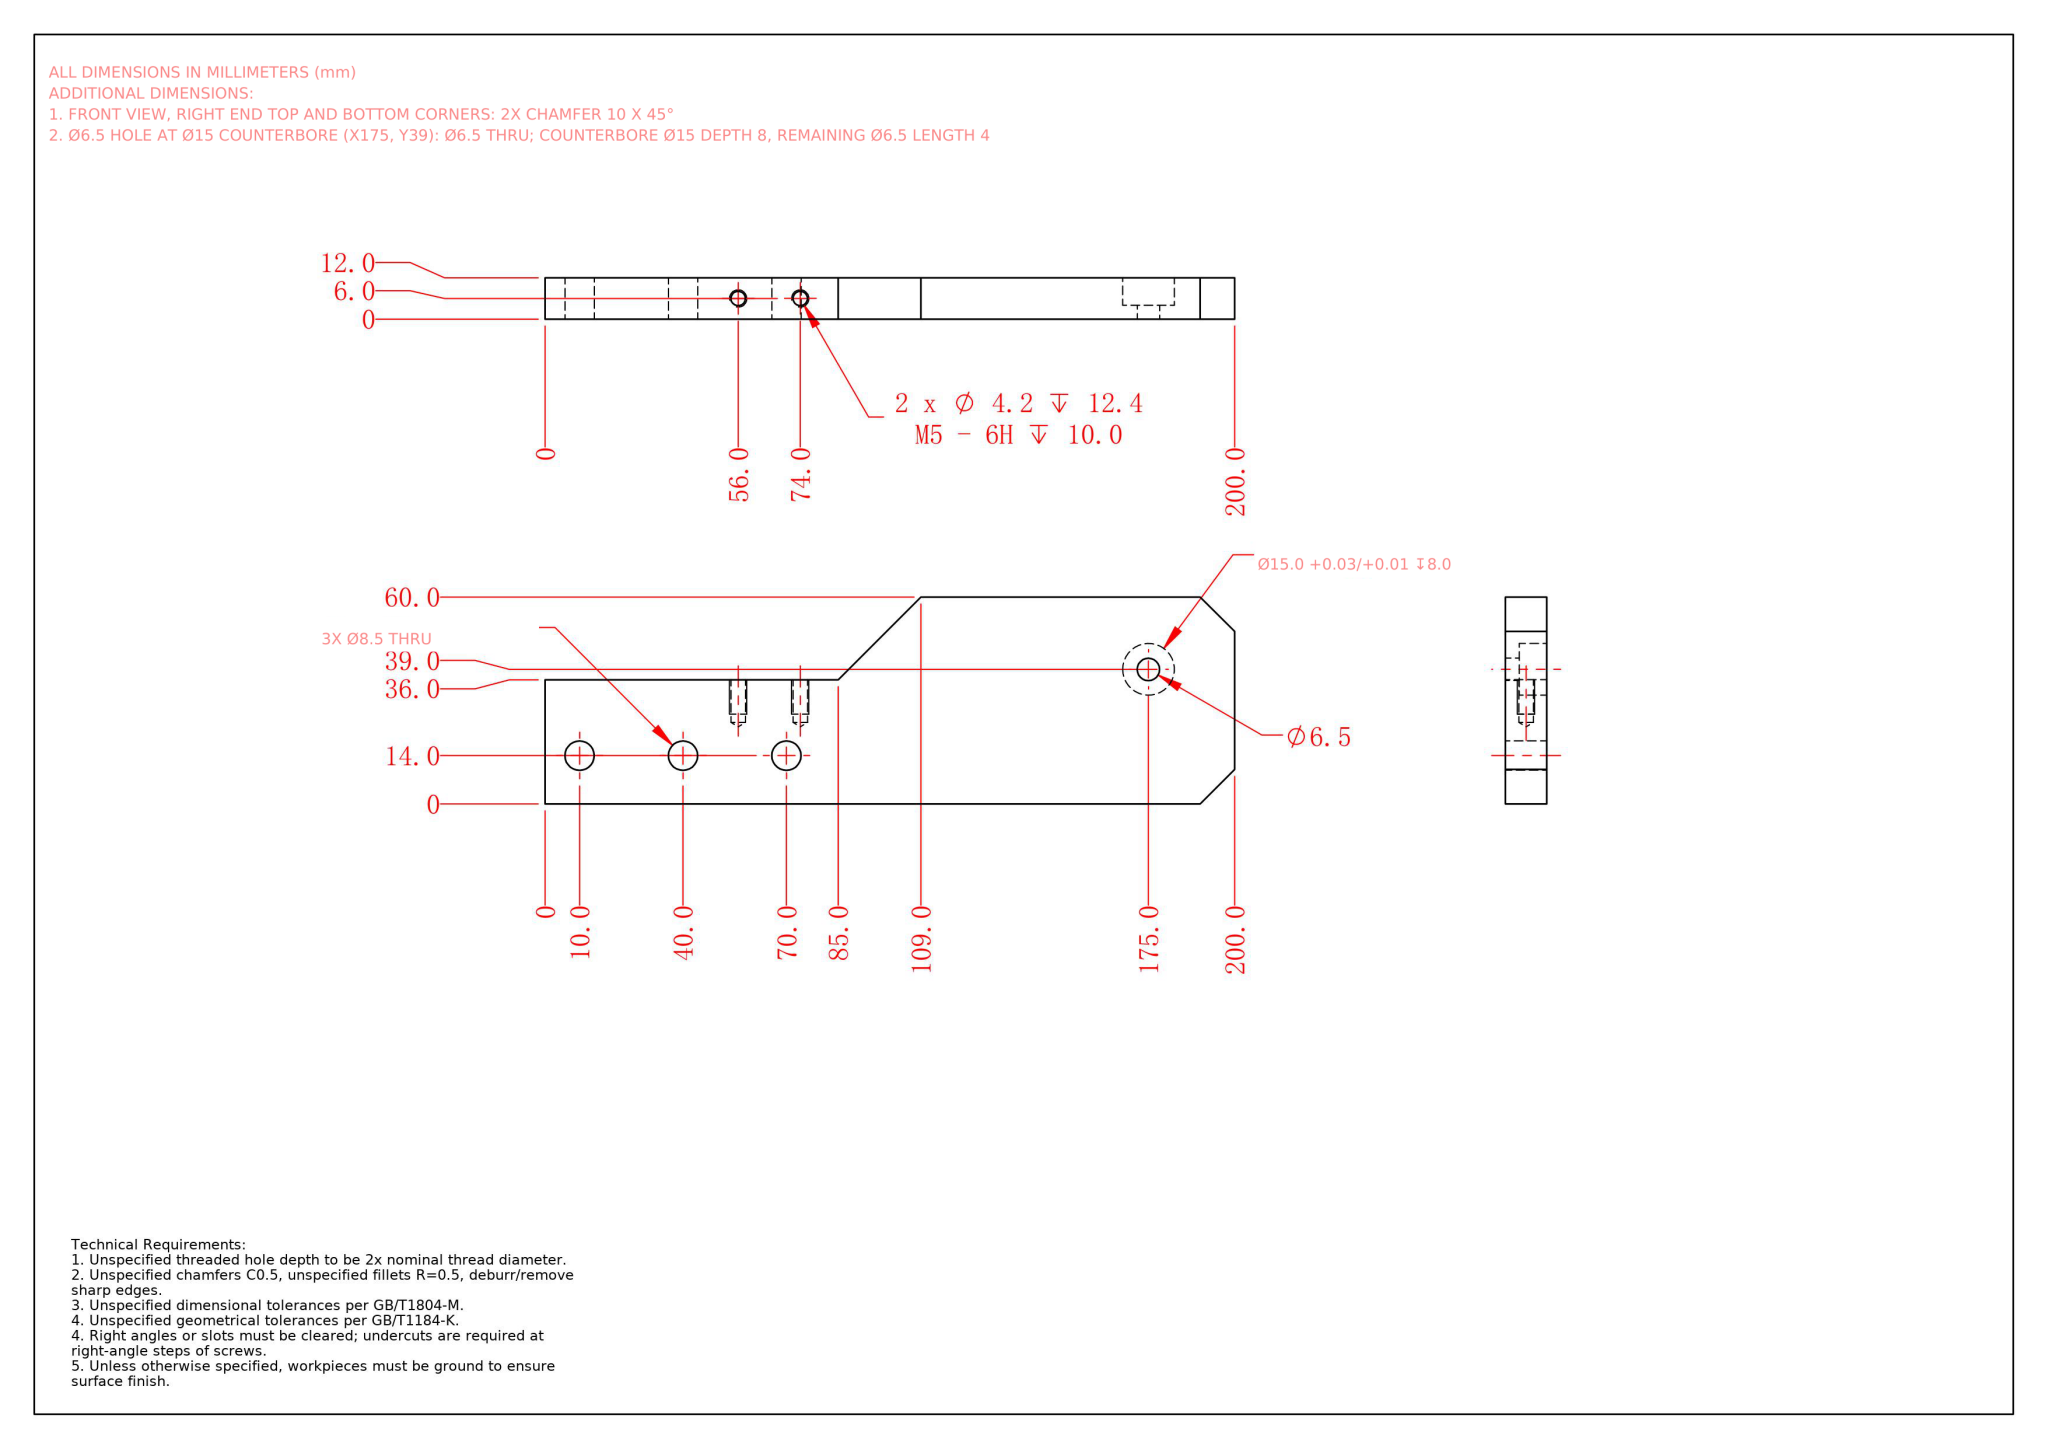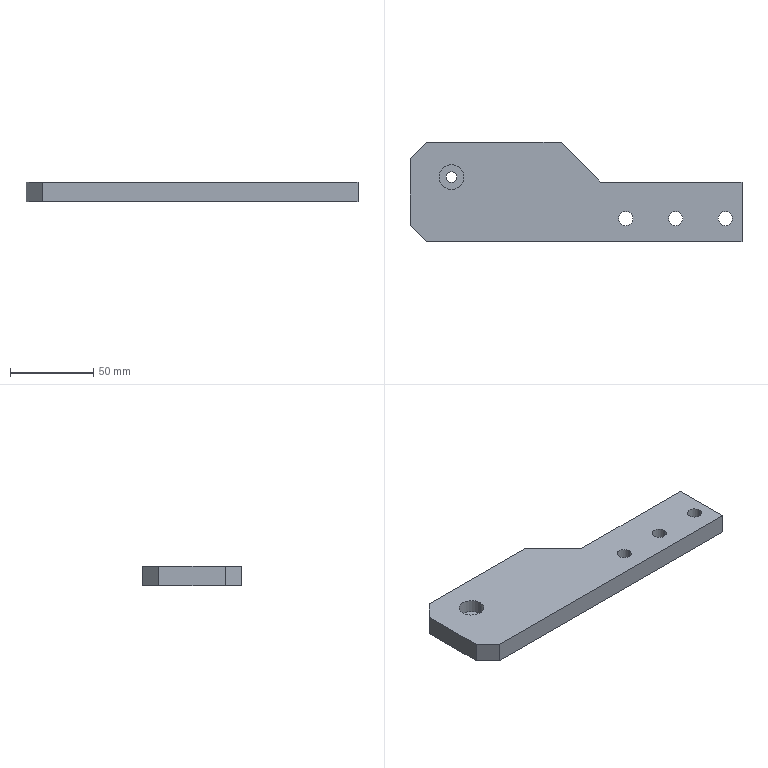Part | NX | mm | 1 solid | 29 faces | box 200 x 60 x 12 mm | volume 110919 mm3 | cylinder 14 | plane 11 | cone 4 | commonest cylinder face diameters 8.5 x6 4.2 x4 6.5 x2 15 x2
STEP:
#1=COLOUR_RGB('',1.,1.,1.);
#2=FILL_AREA_STYLE_COLOUR('',#1);
#3=FILL_AREA_STYLE('',(#2));
#4=SURFACE_STYLE_FILL_AREA(#3);
#5=SURFACE_SIDE_STYLE('',(#4));
#6=SURFACE_STYLE_USAGE(.BOTH.,#5);
#7=PRESENTATION_STYLE_ASSIGNMENT((#6));
#8=CARTESIAN_POINT('',(26.,-6.4,3.9));
#9=VERTEX_POINT('',#8);
#10=CARTESIAN_POINT('',(26.,6.,3.9));
#11=VERTEX_POINT('',#10);
#12=CARTESIAN_POINT('',(26.,6.,3.9));
#13=DIRECTION('',(0.,1.,0.));
#14=VECTOR('',#13,1000.);
#15=LINE('',#12,#14);
#16=EDGE_CURVE('',#9,#11,#15,.T.);
#17=ORIENTED_EDGE('',*,*,#16,.F.);
#18=CARTESIAN_POINT('',(26.,-6.4,8.1));
#19=VERTEX_POINT('',#18);
#20=CARTESIAN_POINT('',(26.,-6.4,6.));
#21=DIRECTION('',(0.,1.,0.));
#22=DIRECTION('',(0.,0.,1.));
#23=AXIS2_PLACEMENT_3D('',#20,#21,#22);
#24=CIRCLE('',#23,2.1);
#25=EDGE_CURVE('',#19,#9,#24,.T.);
#26=ORIENTED_EDGE('',*,*,#25,.F.);
#27=CARTESIAN_POINT('',(26.,6.,8.1));
#28=VERTEX_POINT('',#27);
#29=CARTESIAN_POINT('',(26.,6.,8.1));
#30=DIRECTION('',(0.,1.,0.));
#31=VECTOR('',#30,1000.);
#32=LINE('',#29,#31);
#33=EDGE_CURVE('',#19,#28,#32,.T.);
#34=ORIENTED_EDGE('',*,*,#33,.T.);
#35=CARTESIAN_POINT('',(26.,6.,6.));
#36=DIRECTION('',(0.,1.,0.));
#37=DIRECTION('',(0.,0.,1.));
#38=AXIS2_PLACEMENT_3D('',#35,#36,#37);
#39=CIRCLE('',#38,2.1);
#40=EDGE_CURVE('',#28,#11,#39,.T.);
#41=ORIENTED_EDGE('',*,*,#40,.T.);
#42=EDGE_LOOP('',(#17,#26,#34,#41));
#43=FACE_OUTER_BOUND('',#42,.T.);
#44=CARTESIAN_POINT('',(26.,6.,6.));
#45=DIRECTION('',(0.,1.,0.));
#46=DIRECTION('',(0.,0.,1.));
#47=AXIS2_PLACEMENT_3D('',#44,#45,#46);
#48=CYLINDRICAL_SURFACE('',#47,2.1);
#49=ADVANCED_FACE('',(#43),#48,.F.);
#50=STYLED_ITEM('',(#7),#49);
#51=(LENGTH_UNIT()NAMED_UNIT(*)SI_UNIT(.MILLI.,.METRE.));
#52=UNCERTAINTY_MEASURE_WITH_UNIT(LENGTH_MEASURE(0.00001),#51,'','');
#53=(NAMED_UNIT(*)PLANE_ANGLE_UNIT()SI_UNIT($,.RADIAN.));
#54=(NAMED_UNIT(*)SI_UNIT($,.STERADIAN.)SOLID_ANGLE_UNIT());
#55=(GEOMETRIC_REPRESENTATION_CONTEXT(3)GLOBAL_UNCERTAINTY_ASSIGNED_CONTEXT((#52))GLOBAL_UNIT_ASSIGNED_CONTEXT((#51,#53,#54))REPRESENTATION_CONTEXT('',''));
#56=MECHANICAL_DESIGN_GEOMETRIC_PRESENTATION_REPRESENTATION('',(#50),#55);
#57=COLOUR_RGB('',1.,1.,1.);
#58=FILL_AREA_STYLE_COLOUR('',#57);
#59=FILL_AREA_STYLE('',(#58));
#60=SURFACE_STYLE_FILL_AREA(#59);
#61=SURFACE_SIDE_STYLE('',(#60));
#62=SURFACE_STYLE_USAGE(.BOTH.,#61);
#63=PRESENTATION_STYLE_ASSIGNMENT((#62));
#64=CARTESIAN_POINT('',(44.,-6.4,3.9));
#65=VERTEX_POINT('',#64);
#66=CARTESIAN_POINT('',(44.,-6.4,8.1));
#67=VERTEX_POINT('',#66);
#68=CARTESIAN_POINT('',(44.,-6.4,6.));
#69=DIRECTION('',(0.,1.,0.));
#70=DIRECTION('',(0.,0.,1.));
#71=AXIS2_PLACEMENT_3D('',#68,#69,#70);
#72=CIRCLE('',#71,2.1);
#73=EDGE_CURVE('',#65,#67,#72,.T.);
#74=ORIENTED_EDGE('',*,*,#73,.F.);
#75=CARTESIAN_POINT('',(44.,6.,3.9));
#76=VERTEX_POINT('',#75);
#77=CARTESIAN_POINT('',(44.,6.,3.9));
#78=DIRECTION('',(0.,1.,0.));
#79=VECTOR('',#78,1000.);
#80=LINE('',#77,#79);
#81=EDGE_CURVE('',#65,#76,#80,.T.);
#82=ORIENTED_EDGE('',*,*,#81,.T.);
#83=CARTESIAN_POINT('',(44.,6.,8.1));
#84=VERTEX_POINT('',#83);
#85=CARTESIAN_POINT('',(44.,6.,6.));
#86=DIRECTION('',(0.,1.,0.));
#87=DIRECTION('',(0.,0.,1.));
#88=AXIS2_PLACEMENT_3D('',#85,#86,#87);
#89=CIRCLE('',#88,2.1);
#90=EDGE_CURVE('',#76,#84,#89,.T.);
#91=ORIENTED_EDGE('',*,*,#90,.T.);
#92=CARTESIAN_POINT('',(44.,6.,8.1));
#93=DIRECTION('',(0.,1.,0.));
#94=VECTOR('',#93,1000.);
#95=LINE('',#92,#94);
#96=EDGE_CURVE('',#67,#84,#95,.T.);
#97=ORIENTED_EDGE('',*,*,#96,.F.);
#98=EDGE_LOOP('',(#74,#82,#91,#97));
#99=FACE_OUTER_BOUND('',#98,.T.);
#100=CARTESIAN_POINT('',(44.,6.,6.));
#101=DIRECTION('',(0.,1.,0.));
#102=DIRECTION('',(0.,0.,1.));
#103=AXIS2_PLACEMENT_3D('',#100,#101,#102);
#104=CYLINDRICAL_SURFACE('',#103,2.1);
#105=ADVANCED_FACE('',(#99),#104,.F.);
#106=CARTESIAN_POINT('',(44.,-7.662,6.));
#107=VERTEX_POINT('',#106);
#108=CARTESIAN_POINT('',(44.,-6.4,8.1));
#109=DIRECTION('',(0.,0.515,0.8572));
#110=VECTOR('',#109,1000.);
#111=LINE('',#108,#110);
#112=EDGE_CURVE('',#107,#67,#111,.T.);
#113=ORIENTED_EDGE('',*,*,#112,.F.);
#114=CARTESIAN_POINT('',(44.,-6.4,3.9));
#115=DIRECTION('',(0.,0.515,-0.8572));
#116=VECTOR('',#115,1000.);
#117=LINE('',#114,#116);
#118=EDGE_CURVE('',#107,#65,#117,.T.);
#119=ORIENTED_EDGE('',*,*,#118,.T.);
#120=ORIENTED_EDGE('',*,*,#73,.T.);
#121=EDGE_LOOP('',(#113,#119,#120));
#122=FACE_OUTER_BOUND('',#121,.T.);
#123=CARTESIAN_POINT('',(44.,-6.4,6.));
#124=DIRECTION('',(0.,1.,0.));
#125=DIRECTION('',(0.,0.,1.));
#126=AXIS2_PLACEMENT_3D('',#123,#124,#125);
#127=CONICAL_SURFACE('',#126,2.1,1.03);
#128=ADVANCED_FACE('',(#122),#127,.F.);
#129=CARTESIAN_POINT('',(26.,-6.4,6.));
#130=DIRECTION('',(0.,1.,0.));
#131=DIRECTION('',(0.,0.,1.));
#132=AXIS2_PLACEMENT_3D('',#129,#130,#131);
#133=CIRCLE('',#132,2.1);
#134=EDGE_CURVE('',#9,#19,#133,.T.);
#135=ORIENTED_EDGE('',*,*,#134,.F.);
#136=ORIENTED_EDGE('',*,*,#16,.T.);
#137=CARTESIAN_POINT('',(26.,6.,6.));
#138=DIRECTION('',(0.,1.,0.));
#139=DIRECTION('',(0.,0.,1.));
#140=AXIS2_PLACEMENT_3D('',#137,#138,#139);
#141=CIRCLE('',#140,2.1);
#142=EDGE_CURVE('',#11,#28,#141,.T.);
#143=ORIENTED_EDGE('',*,*,#142,.T.);
#144=ORIENTED_EDGE('',*,*,#33,.F.);
#145=EDGE_LOOP('',(#135,#136,#143,#144));
#146=FACE_OUTER_BOUND('',#145,.T.);
#147=CARTESIAN_POINT('',(26.,6.,6.));
#148=DIRECTION('',(0.,1.,0.));
#149=DIRECTION('',(0.,0.,1.));
#150=AXIS2_PLACEMENT_3D('',#147,#148,#149);
#151=CYLINDRICAL_SURFACE('',#150,2.1);
#152=ADVANCED_FACE('',(#146),#151,.F.);
#153=CARTESIAN_POINT('',(26.,-7.662,6.));
#154=VERTEX_POINT('',#153);
#155=CARTESIAN_POINT('',(26.,-6.4,8.1));
#156=DIRECTION('',(0.,0.515,0.8572));
#157=VECTOR('',#156,1000.);
#158=LINE('',#155,#157);
#159=EDGE_CURVE('',#154,#19,#158,.T.);
#160=ORIENTED_EDGE('',*,*,#159,.F.);
#161=CARTESIAN_POINT('',(26.,-6.4,3.9));
#162=DIRECTION('',(0.,0.515,-0.8572));
#163=VECTOR('',#162,1000.);
#164=LINE('',#161,#163);
#165=EDGE_CURVE('',#154,#9,#164,.T.);
#166=ORIENTED_EDGE('',*,*,#165,.T.);
#167=ORIENTED_EDGE('',*,*,#134,.T.);
#168=EDGE_LOOP('',(#160,#166,#167));
#169=FACE_OUTER_BOUND('',#168,.T.);
#170=CARTESIAN_POINT('',(26.,-6.4,6.));
#171=DIRECTION('',(0.,1.,0.));
#172=DIRECTION('',(0.,0.,1.));
#173=AXIS2_PLACEMENT_3D('',#170,#171,#172);
#174=CONICAL_SURFACE('',#173,2.1,1.03);
#175=ADVANCED_FACE('',(#169),#174,.F.);
#176=CARTESIAN_POINT('',(85.75,-16.,12.));
#177=VERTEX_POINT('',#176);
#178=CARTESIAN_POINT('',(94.25,-16.,12.));
#179=VERTEX_POINT('',#178);
#180=CARTESIAN_POINT('',(90.,-16.,12.));
#181=DIRECTION('',(0.,0.,1.));
#182=DIRECTION('',(1.,0.,0.));
#183=AXIS2_PLACEMENT_3D('',#180,#181,#182);
#184=CIRCLE('',#183,4.25);
#185=EDGE_CURVE('',#177,#179,#184,.T.);
#186=ORIENTED_EDGE('',*,*,#185,.T.);
#187=CARTESIAN_POINT('',(94.25,-16.,0.));
#188=VERTEX_POINT('',#187);
#189=CARTESIAN_POINT('',(94.25,-16.,0.));
#190=DIRECTION('',(0.,0.,-1.));
#191=VECTOR('',#190,1000.);
#192=LINE('',#189,#191);
#193=EDGE_CURVE('',#179,#188,#192,.T.);
#194=ORIENTED_EDGE('',*,*,#193,.T.);
#195=CARTESIAN_POINT('',(85.75,-16.,0.));
#196=VERTEX_POINT('',#195);
#197=CARTESIAN_POINT('',(90.,-16.,0.));
#198=DIRECTION('',(0.,0.,-1.));
#199=DIRECTION('',(-1.,0.,0.));
#200=AXIS2_PLACEMENT_3D('',#197,#198,#199);
#201=CIRCLE('',#200,4.25);
#202=EDGE_CURVE('',#188,#196,#201,.T.);
#203=ORIENTED_EDGE('',*,*,#202,.T.);
#204=CARTESIAN_POINT('',(85.75,-16.,0.));
#205=DIRECTION('',(0.,0.,-1.));
#206=VECTOR('',#205,1000.);
#207=LINE('',#204,#206);
#208=EDGE_CURVE('',#177,#196,#207,.T.);
#209=ORIENTED_EDGE('',*,*,#208,.F.);
#210=EDGE_LOOP('',(#186,#194,#203,#209));
#211=FACE_OUTER_BOUND('',#210,.T.);
#212=CARTESIAN_POINT('',(90.,-16.,0.));
#213=DIRECTION('',(0.,0.,-1.));
#214=DIRECTION('',(-1.,0.,0.));
#215=AXIS2_PLACEMENT_3D('',#212,#213,#214);
#216=CYLINDRICAL_SURFACE('',#215,4.25);
#217=ADVANCED_FACE('',(#211),#216,.F.);
#218=CARTESIAN_POINT('',(55.75,-16.,12.));
#219=VERTEX_POINT('',#218);
#220=CARTESIAN_POINT('',(64.25,-16.,12.));
#221=VERTEX_POINT('',#220);
#222=CARTESIAN_POINT('',(60.,-16.,12.));
#223=DIRECTION('',(0.,0.,1.));
#224=DIRECTION('',(1.,0.,0.));
#225=AXIS2_PLACEMENT_3D('',#222,#223,#224);
#226=CIRCLE('',#225,4.25);
#227=EDGE_CURVE('',#219,#221,#226,.T.);
#228=ORIENTED_EDGE('',*,*,#227,.T.);
#229=CARTESIAN_POINT('',(64.25,-16.,0.));
#230=VERTEX_POINT('',#229);
#231=CARTESIAN_POINT('',(64.25,-16.,0.));
#232=DIRECTION('',(0.,0.,-1.));
#233=VECTOR('',#232,1000.);
#234=LINE('',#231,#233);
#235=EDGE_CURVE('',#221,#230,#234,.T.);
#236=ORIENTED_EDGE('',*,*,#235,.T.);
#237=CARTESIAN_POINT('',(55.75,-16.,0.));
#238=VERTEX_POINT('',#237);
#239=CARTESIAN_POINT('',(60.,-16.,0.));
#240=DIRECTION('',(0.,0.,-1.));
#241=DIRECTION('',(-1.,0.,0.));
#242=AXIS2_PLACEMENT_3D('',#239,#240,#241);
#243=CIRCLE('',#242,4.25);
#244=EDGE_CURVE('',#230,#238,#243,.T.);
#245=ORIENTED_EDGE('',*,*,#244,.T.);
#246=CARTESIAN_POINT('',(55.75,-16.,0.));
#247=DIRECTION('',(0.,0.,-1.));
#248=VECTOR('',#247,1000.);
#249=LINE('',#246,#248);
#250=EDGE_CURVE('',#219,#238,#249,.T.);
#251=ORIENTED_EDGE('',*,*,#250,.F.);
#252=EDGE_LOOP('',(#228,#236,#245,#251));
#253=FACE_OUTER_BOUND('',#252,.T.);
#254=CARTESIAN_POINT('',(60.,-16.,0.));
#255=DIRECTION('',(0.,0.,-1.));
#256=DIRECTION('',(-1.,0.,0.));
#257=AXIS2_PLACEMENT_3D('',#254,#255,#256);
#258=CYLINDRICAL_SURFACE('',#257,4.25);
#259=ADVANCED_FACE('',(#253),#258,.F.);
#260=CARTESIAN_POINT('',(25.75,-16.,12.));
#261=VERTEX_POINT('',#260);
#262=CARTESIAN_POINT('',(34.25,-16.,12.));
#263=VERTEX_POINT('',#262);
#264=CARTESIAN_POINT('',(30.,-16.,12.));
#265=DIRECTION('',(0.,0.,1.));
#266=DIRECTION('',(1.,0.,0.));
#267=AXIS2_PLACEMENT_3D('',#264,#265,#266);
#268=CIRCLE('',#267,4.25);
#269=EDGE_CURVE('',#261,#263,#268,.T.);
#270=ORIENTED_EDGE('',*,*,#269,.T.);
#271=CARTESIAN_POINT('',(34.25,-16.,0.));
#272=VERTEX_POINT('',#271);
#273=CARTESIAN_POINT('',(34.25,-16.,0.));
#274=DIRECTION('',(0.,0.,-1.));
#275=VECTOR('',#274,1000.);
#276=LINE('',#273,#275);
#277=EDGE_CURVE('',#263,#272,#276,.T.);
#278=ORIENTED_EDGE('',*,*,#277,.T.);
#279=CARTESIAN_POINT('',(25.75,-16.,0.));
#280=VERTEX_POINT('',#279);
#281=CARTESIAN_POINT('',(30.,-16.,0.));
#282=DIRECTION('',(0.,0.,-1.));
#283=DIRECTION('',(-1.,0.,0.));
#284=AXIS2_PLACEMENT_3D('',#281,#282,#283);
#285=CIRCLE('',#284,4.25);
#286=EDGE_CURVE('',#272,#280,#285,.T.);
#287=ORIENTED_EDGE('',*,*,#286,.T.);
#288=CARTESIAN_POINT('',(25.75,-16.,0.));
#289=DIRECTION('',(0.,0.,-1.));
#290=VECTOR('',#289,1000.);
#291=LINE('',#288,#290);
#292=EDGE_CURVE('',#261,#280,#291,.T.);
#293=ORIENTED_EDGE('',*,*,#292,.F.);
#294=EDGE_LOOP('',(#270,#278,#287,#293));
#295=FACE_OUTER_BOUND('',#294,.T.);
#296=CARTESIAN_POINT('',(30.,-16.,0.));
#297=DIRECTION('',(0.,0.,-1.));
#298=DIRECTION('',(-1.,0.,0.));
#299=AXIS2_PLACEMENT_3D('',#296,#297,#298);
#300=CYLINDRICAL_SURFACE('',#299,4.25);
#301=ADVANCED_FACE('',(#295),#300,.F.);
#302=CARTESIAN_POINT('',(-71.75,9.,0.));
#303=VERTEX_POINT('',#302);
#304=CARTESIAN_POINT('',(-78.25,9.,0.));
#305=VERTEX_POINT('',#304);
#306=CARTESIAN_POINT('',(-75.,9.,0.));
#307=DIRECTION('',(0.,0.,-1.));
#308=DIRECTION('',(1.,0.,0.));
#309=AXIS2_PLACEMENT_3D('',#306,#307,#308);
#310=CIRCLE('',#309,3.25);
#311=EDGE_CURVE('',#303,#305,#310,.T.);
#312=ORIENTED_EDGE('',*,*,#311,.T.);
#313=CARTESIAN_POINT('',(-78.25,9.,4.));
#314=VERTEX_POINT('',#313);
#315=CARTESIAN_POINT('',(-78.25,9.,-0.001));
#316=DIRECTION('',(0.,0.,1.));
#317=VECTOR('',#316,1000.);
#318=LINE('',#315,#317);
#319=EDGE_CURVE('',#305,#314,#318,.T.);
#320=ORIENTED_EDGE('',*,*,#319,.T.);
#321=CARTESIAN_POINT('',(-71.75,9.,4.));
#322=VERTEX_POINT('',#321);
#323=CARTESIAN_POINT('',(-75.,9.,4.));
#324=DIRECTION('',(0.,0.,1.));
#325=DIRECTION('',(1.,0.,0.));
#326=AXIS2_PLACEMENT_3D('',#323,#324,#325);
#327=CIRCLE('',#326,3.25);
#328=EDGE_CURVE('',#314,#322,#327,.T.);
#329=ORIENTED_EDGE('',*,*,#328,.T.);
#330=CARTESIAN_POINT('',(-71.75,9.,-0.001));
#331=DIRECTION('',(0.,0.,1.));
#332=VECTOR('',#331,1000.);
#333=LINE('',#330,#332);
#334=EDGE_CURVE('',#303,#322,#333,.T.);
#335=ORIENTED_EDGE('',*,*,#334,.F.);
#336=EDGE_LOOP('',(#312,#320,#329,#335));
#337=FACE_OUTER_BOUND('',#336,.T.);
#338=CARTESIAN_POINT('',(-75.,9.,-0.001));
#339=DIRECTION('',(0.,0.,1.));
#340=DIRECTION('',(1.,0.,0.));
#341=AXIS2_PLACEMENT_3D('',#338,#339,#340);
#342=CYLINDRICAL_SURFACE('',#341,3.25);
#343=ADVANCED_FACE('',(#337),#342,.F.);
#344=CARTESIAN_POINT('',(-82.5,9.,4.));
#345=VERTEX_POINT('',#344);
#346=CARTESIAN_POINT('',(-67.5,9.,4.));
#347=VERTEX_POINT('',#346);
#348=CARTESIAN_POINT('',(-75.,9.,4.));
#349=DIRECTION('',(0.,0.,1.));
#350=DIRECTION('',(1.,0.,0.));
#351=AXIS2_PLACEMENT_3D('',#348,#349,#350);
#352=CIRCLE('',#351,7.5);
#353=EDGE_CURVE('',#345,#347,#352,.T.);
#354=ORIENTED_EDGE('',*,*,#353,.F.);
#355=CARTESIAN_POINT('',(-82.5,9.,12.));
#356=VERTEX_POINT('',#355);
#357=CARTESIAN_POINT('',(-82.5,9.,4.));
#358=DIRECTION('',(0.,0.,1.));
#359=VECTOR('',#358,1000.);
#360=LINE('',#357,#359);
#361=EDGE_CURVE('',#345,#356,#360,.T.);
#362=ORIENTED_EDGE('',*,*,#361,.T.);
#363=CARTESIAN_POINT('',(-67.5,9.,12.));
#364=VERTEX_POINT('',#363);
#365=CARTESIAN_POINT('',(-75.,9.,12.));
#366=DIRECTION('',(0.,0.,1.));
#367=DIRECTION('',(1.,0.,0.));
#368=AXIS2_PLACEMENT_3D('',#365,#366,#367);
#369=CIRCLE('',#368,7.5);
#370=EDGE_CURVE('',#356,#364,#369,.T.);
#371=ORIENTED_EDGE('',*,*,#370,.T.);
#372=CARTESIAN_POINT('',(-67.5,9.,4.));
#373=DIRECTION('',(0.,0.,1.));
#374=VECTOR('',#373,1000.);
#375=LINE('',#372,#374);
#376=EDGE_CURVE('',#347,#364,#375,.T.);
#377=ORIENTED_EDGE('',*,*,#376,.F.);
#378=EDGE_LOOP('',(#354,#362,#371,#377));
#379=FACE_OUTER_BOUND('',#378,.T.);
#380=CARTESIAN_POINT('',(-75.,9.,4.));
#381=DIRECTION('',(0.,0.,1.));
#382=DIRECTION('',(1.,0.,0.));
#383=AXIS2_PLACEMENT_3D('',#380,#381,#382);
#384=CYLINDRICAL_SURFACE('',#383,7.5);
#385=ADVANCED_FACE('',(#379),#384,.F.);
#386=CARTESIAN_POINT('',(60.,-16.,0.));
#387=DIRECTION('',(0.,0.,-1.));
#388=DIRECTION('',(-1.,0.,0.));
#389=AXIS2_PLACEMENT_3D('',#386,#387,#388);
#390=CIRCLE('',#389,4.25);
#391=EDGE_CURVE('',#238,#230,#390,.T.);
#392=ORIENTED_EDGE('',*,*,#391,.F.);
#393=ORIENTED_EDGE('',*,*,#244,.F.);
#394=EDGE_LOOP('',(#392,#393));
#395=FACE_BOUND('',#394,.T.);
#396=CARTESIAN_POINT('',(30.,-16.,0.));
#397=DIRECTION('',(0.,0.,-1.));
#398=DIRECTION('',(-1.,0.,0.));
#399=AXIS2_PLACEMENT_3D('',#396,#397,#398);
#400=CIRCLE('',#399,4.25);
#401=EDGE_CURVE('',#280,#272,#400,.T.);
#402=ORIENTED_EDGE('',*,*,#401,.F.);
#403=ORIENTED_EDGE('',*,*,#286,.F.);
#404=EDGE_LOOP('',(#402,#403));
#405=FACE_BOUND('',#404,.T.);
#406=ORIENTED_EDGE('',*,*,#311,.F.);
#407=CARTESIAN_POINT('',(-75.,9.,0.));
#408=DIRECTION('',(0.,0.,-1.));
#409=DIRECTION('',(1.,0.,0.));
#410=AXIS2_PLACEMENT_3D('',#407,#408,#409);
#411=CIRCLE('',#410,3.25);
#412=EDGE_CURVE('',#305,#303,#411,.T.);
#413=ORIENTED_EDGE('',*,*,#412,.F.);
#414=EDGE_LOOP('',(#406,#413));
#415=FACE_BOUND('',#414,.T.);
#416=CARTESIAN_POINT('',(-9.,30.,0.));
#417=VERTEX_POINT('',#416);
#418=CARTESIAN_POINT('',(-90.,30.,0.));
#419=VERTEX_POINT('',#418);
#420=CARTESIAN_POINT('',(-100.,30.,0.));
#421=DIRECTION('',(-1.,0.,0.));
#422=VECTOR('',#421,1000.);
#423=LINE('',#420,#422);
#424=EDGE_CURVE('',#417,#419,#423,.T.);
#425=ORIENTED_EDGE('',*,*,#424,.F.);
#426=CARTESIAN_POINT('',(15.,6.,0.));
#427=VERTEX_POINT('',#426);
#428=CARTESIAN_POINT('',(-9.,30.,0.));
#429=DIRECTION('',(0.7071,-0.7071,0.));
#430=VECTOR('',#429,1000.);
#431=LINE('',#428,#430);
#432=EDGE_CURVE('',#417,#427,#431,.T.);
#433=ORIENTED_EDGE('',*,*,#432,.T.);
#434=CARTESIAN_POINT('',(100.,6.,0.));
#435=VERTEX_POINT('',#434);
#436=CARTESIAN_POINT('',(100.,6.,0.));
#437=DIRECTION('',(-1.,0.,0.));
#438=VECTOR('',#437,1000.);
#439=LINE('',#436,#438);
#440=EDGE_CURVE('',#435,#427,#439,.T.);
#441=ORIENTED_EDGE('',*,*,#440,.F.);
#442=CARTESIAN_POINT('',(100.,-30.,0.));
#443=VERTEX_POINT('',#442);
#444=CARTESIAN_POINT('',(100.,30.,0.));
#445=DIRECTION('',(0.,1.,0.));
#446=VECTOR('',#445,1000.);
#447=LINE('',#444,#446);
#448=EDGE_CURVE('',#443,#435,#447,.T.);
#449=ORIENTED_EDGE('',*,*,#448,.F.);
#450=CARTESIAN_POINT('',(-90.,-30.,0.));
#451=VERTEX_POINT('',#450);
#452=CARTESIAN_POINT('',(-100.,-30.,0.));
#453=DIRECTION('',(1.,0.,0.));
#454=VECTOR('',#453,1000.);
#455=LINE('',#452,#454);
#456=EDGE_CURVE('',#451,#443,#455,.T.);
#457=ORIENTED_EDGE('',*,*,#456,.F.);
#458=CARTESIAN_POINT('',(-100.,-20.,0.));
#459=VERTEX_POINT('',#458);
#460=CARTESIAN_POINT('',(-90.,-30.,0.));
#461=DIRECTION('',(-0.7071,0.7071,0.));
#462=VECTOR('',#461,1000.);
#463=LINE('',#460,#462);
#464=EDGE_CURVE('',#451,#459,#463,.T.);
#465=ORIENTED_EDGE('',*,*,#464,.T.);
#466=CARTESIAN_POINT('',(-100.,20.,0.));
#467=VERTEX_POINT('',#466);
#468=CARTESIAN_POINT('',(-100.,30.,0.));
#469=DIRECTION('',(0.,-1.,0.));
#470=VECTOR('',#469,1000.);
#471=LINE('',#468,#470);
#472=EDGE_CURVE('',#467,#459,#471,.T.);
#473=ORIENTED_EDGE('',*,*,#472,.F.);
#474=CARTESIAN_POINT('',(-100.,20.,0.));
#475=DIRECTION('',(0.7071,0.7071,0.));
#476=VECTOR('',#475,1000.);
#477=LINE('',#474,#476);
#478=EDGE_CURVE('',#467,#419,#477,.T.);
#479=ORIENTED_EDGE('',*,*,#478,.T.);
#480=EDGE_LOOP('',(#425,#433,#441,#449,#457,#465,#473,#479));
#481=FACE_OUTER_BOUND('',#480,.T.);
#482=CARTESIAN_POINT('',(90.,-16.,0.));
#483=DIRECTION('',(0.,0.,-1.));
#484=DIRECTION('',(-1.,0.,0.));
#485=AXIS2_PLACEMENT_3D('',#482,#483,#484);
#486=CIRCLE('',#485,4.25);
#487=EDGE_CURVE('',#196,#188,#486,.T.);
#488=ORIENTED_EDGE('',*,*,#487,.F.);
#489=ORIENTED_EDGE('',*,*,#202,.F.);
#490=EDGE_LOOP('',(#488,#489));
#491=FACE_BOUND('',#490,.T.);
#492=CARTESIAN_POINT('',(0.,0.,0.));
#493=DIRECTION('',(0.,0.,1.));
#494=DIRECTION('',(1.,0.,0.));
#495=AXIS2_PLACEMENT_3D('',#492,#493,#494);
#496=PLANE('',#495);
#497=ADVANCED_FACE('',(#395,#405,#415,#481,#491),#496,.F.);
#498=ORIENTED_EDGE('',*,*,#448,.T.);
#499=CARTESIAN_POINT('',(100.,6.,12.));
#500=VERTEX_POINT('',#499);
#501=CARTESIAN_POINT('',(100.,6.,12.001));
#502=DIRECTION('',(0.,0.,-1.));
#503=VECTOR('',#502,1000.);
#504=LINE('',#501,#503);
#505=EDGE_CURVE('',#500,#435,#504,.T.);
#506=ORIENTED_EDGE('',*,*,#505,.F.);
#507=CARTESIAN_POINT('',(100.,-30.,12.));
#508=VERTEX_POINT('',#507);
#509=CARTESIAN_POINT('',(100.,30.,12.));
#510=DIRECTION('',(0.,1.,0.));
#511=VECTOR('',#510,1000.);
#512=LINE('',#509,#511);
#513=EDGE_CURVE('',#508,#500,#512,.T.);
#514=ORIENTED_EDGE('',*,*,#513,.F.);
#515=CARTESIAN_POINT('',(100.,-30.,12.));
#516=DIRECTION('',(0.,0.,-1.));
#517=VECTOR('',#516,1000.);
#518=LINE('',#515,#517);
#519=EDGE_CURVE('',#508,#443,#518,.T.);
#520=ORIENTED_EDGE('',*,*,#519,.T.);
#521=EDGE_LOOP('',(#498,#506,#514,#520));
#522=FACE_OUTER_BOUND('',#521,.T.);
#523=CARTESIAN_POINT('',(100.,30.,12.));
#524=DIRECTION('',(-1.,0.,0.));
#525=DIRECTION('',(0.,0.,1.));
#526=AXIS2_PLACEMENT_3D('',#523,#524,#525);
#527=PLANE('',#526);
#528=ADVANCED_FACE('',(#522),#527,.F.);
#529=CARTESIAN_POINT('',(-9.,30.,12.));
#530=VERTEX_POINT('',#529);
#531=CARTESIAN_POINT('',(-90.,30.,12.));
#532=VERTEX_POINT('',#531);
#533=CARTESIAN_POINT('',(-100.,30.,12.));
#534=DIRECTION('',(-1.,0.,0.));
#535=VECTOR('',#534,1000.);
#536=LINE('',#533,#535);
#537=EDGE_CURVE('',#530,#532,#536,.T.);
#538=ORIENTED_EDGE('',*,*,#537,.F.);
#539=CARTESIAN_POINT('',(-9.,30.,12.));
#540=DIRECTION('',(0.,0.,-1.));
#541=VECTOR('',#540,1000.);
#542=LINE('',#539,#541);
#543=EDGE_CURVE('',#530,#417,#542,.T.);
#544=ORIENTED_EDGE('',*,*,#543,.T.);
#545=ORIENTED_EDGE('',*,*,#424,.T.);
#546=CARTESIAN_POINT('',(-90.,30.,12.));
#547=DIRECTION('',(0.,0.,1.));
#548=VECTOR('',#547,1000.);
#549=LINE('',#546,#548);
#550=EDGE_CURVE('',#419,#532,#549,.T.);
#551=ORIENTED_EDGE('',*,*,#550,.T.);
#552=EDGE_LOOP('',(#538,#544,#545,#551));
#553=FACE_OUTER_BOUND('',#552,.T.);
#554=CARTESIAN_POINT('',(-100.,30.,12.));
#555=DIRECTION('',(0.,-1.,0.));
#556=DIRECTION('',(0.,0.,-1.));
#557=AXIS2_PLACEMENT_3D('',#554,#555,#556);
#558=PLANE('',#557);
#559=ADVANCED_FACE('',(#553),#558,.F.);
#560=ORIENTED_EDGE('',*,*,#472,.T.);
#561=CARTESIAN_POINT('',(-100.,-20.,12.));
#562=VERTEX_POINT('',#561);
#563=CARTESIAN_POINT('',(-100.,-20.,12.));
#564=DIRECTION('',(0.,0.,1.));
#565=VECTOR('',#564,1000.);
#566=LINE('',#563,#565);
#567=EDGE_CURVE('',#459,#562,#566,.T.);
#568=ORIENTED_EDGE('',*,*,#567,.T.);
#569=CARTESIAN_POINT('',(-100.,20.,12.));
#570=VERTEX_POINT('',#569);
#571=CARTESIAN_POINT('',(-100.,30.,12.));
#572=DIRECTION('',(0.,-1.,0.));
#573=VECTOR('',#572,1000.);
#574=LINE('',#571,#573);
#575=EDGE_CURVE('',#570,#562,#574,.T.);
#576=ORIENTED_EDGE('',*,*,#575,.F.);
#577=CARTESIAN_POINT('',(-100.,20.,12.));
#578=DIRECTION('',(0.,0.,-1.));
#579=VECTOR('',#578,1000.);
#580=LINE('',#577,#579);
#581=EDGE_CURVE('',#570,#467,#580,.T.);
#582=ORIENTED_EDGE('',*,*,#581,.T.);
#583=EDGE_LOOP('',(#560,#568,#576,#582));
#584=FACE_OUTER_BOUND('',#583,.T.);
#585=CARTESIAN_POINT('',(-100.,30.,12.));
#586=DIRECTION('',(1.,0.,0.));
#587=DIRECTION('',(0.,0.,-1.));
#588=AXIS2_PLACEMENT_3D('',#585,#586,#587);
#589=PLANE('',#588);
#590=ADVANCED_FACE('',(#584),#589,.F.);
#591=CARTESIAN_POINT('',(-90.,-30.,12.));
#592=VERTEX_POINT('',#591);
#593=CARTESIAN_POINT('',(-100.,-30.,12.));
#594=DIRECTION('',(1.,0.,0.));
#595=VECTOR('',#594,1000.);
#596=LINE('',#593,#595);
#597=EDGE_CURVE('',#592,#508,#596,.T.);
#598=ORIENTED_EDGE('',*,*,#597,.F.);
#599=CARTESIAN_POINT('',(-90.,-30.,12.));
#600=DIRECTION('',(0.,0.,-1.));
#601=VECTOR('',#600,1000.);
#602=LINE('',#599,#601);
#603=EDGE_CURVE('',#592,#451,#602,.T.);
#604=ORIENTED_EDGE('',*,*,#603,.T.);
#605=ORIENTED_EDGE('',*,*,#456,.T.);
#606=ORIENTED_EDGE('',*,*,#519,.F.);
#607=EDGE_LOOP('',(#598,#604,#605,#606));
#608=FACE_OUTER_BOUND('',#607,.T.);
#609=CARTESIAN_POINT('',(-100.,-30.,12.));
#610=DIRECTION('',(0.,1.,0.));
#611=DIRECTION('',(0.,0.,1.));
#612=AXIS2_PLACEMENT_3D('',#609,#610,#611);
#613=PLANE('',#612);
#614=ADVANCED_FACE('',(#608),#613,.F.);
#615=CARTESIAN_POINT('',(15.,6.,12.));
#616=VERTEX_POINT('',#615);
#617=CARTESIAN_POINT('',(100.,6.,12.));
#618=DIRECTION('',(-1.,0.,0.));
#619=VECTOR('',#618,1000.);
#620=LINE('',#617,#619);
#621=EDGE_CURVE('',#500,#616,#620,.T.);
#622=ORIENTED_EDGE('',*,*,#621,.T.);
#623=CARTESIAN_POINT('',(10.5,10.5,12.));
#624=DIRECTION('',(-0.7071,0.7071,0.));
#625=VECTOR('',#624,1000.);
#626=LINE('',#623,#625);
#627=EDGE_CURVE('',#616,#530,#626,.T.);
#628=ORIENTED_EDGE('',*,*,#627,.T.);
#629=ORIENTED_EDGE('',*,*,#537,.T.);
#630=CARTESIAN_POINT('',(-60.,60.,12.));
#631=DIRECTION('',(-0.7071,-0.7071,0.));
#632=VECTOR('',#631,1000.);
#633=LINE('',#630,#632);
#634=EDGE_CURVE('',#532,#570,#633,.T.);
#635=ORIENTED_EDGE('',*,*,#634,.T.);
#636=ORIENTED_EDGE('',*,*,#575,.T.);
#637=CARTESIAN_POINT('',(-60.,-60.,12.));
#638=DIRECTION('',(0.7071,-0.7071,0.));
#639=VECTOR('',#638,1000.);
#640=LINE('',#637,#639);
#641=EDGE_CURVE('',#562,#592,#640,.T.);
#642=ORIENTED_EDGE('',*,*,#641,.T.);
#643=ORIENTED_EDGE('',*,*,#597,.T.);
#644=ORIENTED_EDGE('',*,*,#513,.T.);
#645=EDGE_LOOP('',(#622,#628,#629,#635,#636,#642,#643,#644));
#646=FACE_OUTER_BOUND('',#645,.T.);
#647=ORIENTED_EDGE('',*,*,#185,.F.);
#648=CARTESIAN_POINT('',(90.,-16.,12.));
#649=DIRECTION('',(0.,0.,1.));
#650=DIRECTION('',(1.,0.,0.));
#651=AXIS2_PLACEMENT_3D('',#648,#649,#650);
#652=CIRCLE('',#651,4.25);
#653=EDGE_CURVE('',#179,#177,#652,.T.);
#654=ORIENTED_EDGE('',*,*,#653,.F.);
#655=EDGE_LOOP('',(#647,#654));
#656=FACE_BOUND('',#655,.T.);
#657=ORIENTED_EDGE('',*,*,#227,.F.);
#658=CARTESIAN_POINT('',(60.,-16.,12.));
#659=DIRECTION('',(0.,0.,1.));
#660=DIRECTION('',(1.,0.,0.));
#661=AXIS2_PLACEMENT_3D('',#658,#659,#660);
#662=CIRCLE('',#661,4.25);
#663=EDGE_CURVE('',#221,#219,#662,.T.);
#664=ORIENTED_EDGE('',*,*,#663,.F.);
#665=EDGE_LOOP('',(#657,#664));
#666=FACE_BOUND('',#665,.T.);
#667=ORIENTED_EDGE('',*,*,#269,.F.);
#668=CARTESIAN_POINT('',(30.,-16.,12.));
#669=DIRECTION('',(0.,0.,1.));
#670=DIRECTION('',(1.,0.,0.));
#671=AXIS2_PLACEMENT_3D('',#668,#669,#670);
#672=CIRCLE('',#671,4.25);
#673=EDGE_CURVE('',#263,#261,#672,.T.);
#674=ORIENTED_EDGE('',*,*,#673,.F.);
#675=EDGE_LOOP('',(#667,#674));
#676=FACE_BOUND('',#675,.T.);
#677=CARTESIAN_POINT('',(-75.,9.,12.));
#678=DIRECTION('',(0.,0.,1.));
#679=DIRECTION('',(1.,0.,0.));
#680=AXIS2_PLACEMENT_3D('',#677,#678,#679);
#681=CIRCLE('',#680,7.5);
#682=EDGE_CURVE('',#364,#356,#681,.T.);
#683=ORIENTED_EDGE('',*,*,#682,.F.);
#684=ORIENTED_EDGE('',*,*,#370,.F.);
#685=EDGE_LOOP('',(#683,#684));
#686=FACE_BOUND('',#685,.T.);
#687=CARTESIAN_POINT('',(0.,0.,12.));
#688=DIRECTION('',(0.,0.,1.));
#689=DIRECTION('',(1.,0.,0.));
#690=AXIS2_PLACEMENT_3D('',#687,#688,#689);
#691=PLANE('',#690);
#692=ADVANCED_FACE('',(#646,#656,#666,#676,#686),#691,.T.);
#693=ORIENTED_EDGE('',*,*,#361,.F.);
#694=CARTESIAN_POINT('',(-75.,9.,4.));
#695=DIRECTION('',(0.,0.,1.));
#696=DIRECTION('',(1.,0.,0.));
#697=AXIS2_PLACEMENT_3D('',#694,#695,#696);
#698=CIRCLE('',#697,7.5);
#699=EDGE_CURVE('',#347,#345,#698,.T.);
#700=ORIENTED_EDGE('',*,*,#699,.F.);
#701=ORIENTED_EDGE('',*,*,#376,.T.);
#702=ORIENTED_EDGE('',*,*,#682,.T.);
#703=EDGE_LOOP('',(#693,#700,#701,#702));
#704=FACE_OUTER_BOUND('',#703,.T.);
#705=CARTESIAN_POINT('',(-75.,9.,4.));
#706=DIRECTION('',(0.,0.,1.));
#707=DIRECTION('',(1.,0.,0.));
#708=AXIS2_PLACEMENT_3D('',#705,#706,#707);
#709=CYLINDRICAL_SURFACE('',#708,7.5);
#710=ADVANCED_FACE('',(#704),#709,.F.);
#711=CARTESIAN_POINT('',(-75.,9.,4.));
#712=DIRECTION('',(0.,0.,1.));
#713=DIRECTION('',(1.,0.,0.));
#714=AXIS2_PLACEMENT_3D('',#711,#712,#713);
#715=CIRCLE('',#714,3.25);
#716=EDGE_CURVE('',#322,#314,#715,.T.);
#717=ORIENTED_EDGE('',*,*,#716,.F.);
#718=ORIENTED_EDGE('',*,*,#328,.F.);
#719=EDGE_LOOP('',(#717,#718));
#720=FACE_BOUND('',#719,.T.);
#721=ORIENTED_EDGE('',*,*,#699,.T.);
#722=ORIENTED_EDGE('',*,*,#353,.T.);
#723=EDGE_LOOP('',(#721,#722));
#724=FACE_OUTER_BOUND('',#723,.T.);
#725=CARTESIAN_POINT('',(-75.,9.,4.));
#726=DIRECTION('',(0.,0.,1.));
#727=DIRECTION('',(1.,0.,0.));
#728=AXIS2_PLACEMENT_3D('',#725,#726,#727);
#729=PLANE('',#728);
#730=ADVANCED_FACE('',(#720,#724),#729,.T.);
#731=ORIENTED_EDGE('',*,*,#641,.F.);
#732=ORIENTED_EDGE('',*,*,#567,.F.);
#733=ORIENTED_EDGE('',*,*,#464,.F.);
#734=ORIENTED_EDGE('',*,*,#603,.F.);
#735=EDGE_LOOP('',(#731,#732,#733,#734));
#736=FACE_OUTER_BOUND('',#735,.T.);
#737=CARTESIAN_POINT('',(-90.,-30.,12.));
#738=DIRECTION('',(0.7071,0.7071,0.));
#739=DIRECTION('',(0.,0.,-1.));
#740=AXIS2_PLACEMENT_3D('',#737,#738,#739);
#741=PLANE('',#740);
#742=ADVANCED_FACE('',(#736),#741,.F.);
#743=ORIENTED_EDGE('',*,*,#634,.F.);
#744=ORIENTED_EDGE('',*,*,#550,.F.);
#745=ORIENTED_EDGE('',*,*,#478,.F.);
#746=ORIENTED_EDGE('',*,*,#581,.F.);
#747=EDGE_LOOP('',(#743,#744,#745,#746));
#748=FACE_OUTER_BOUND('',#747,.T.);
#749=CARTESIAN_POINT('',(-100.,20.,12.));
#750=DIRECTION('',(0.7071,-0.7071,0.));
#751=DIRECTION('',(0.,0.,-1.));
#752=AXIS2_PLACEMENT_3D('',#749,#750,#751);
#753=PLANE('',#752);
#754=ADVANCED_FACE('',(#748),#753,.F.);
#755=ORIENTED_EDGE('',*,*,#319,.F.);
#756=ORIENTED_EDGE('',*,*,#412,.T.);
#757=ORIENTED_EDGE('',*,*,#334,.T.);
#758=ORIENTED_EDGE('',*,*,#716,.T.);
#759=EDGE_LOOP('',(#755,#756,#757,#758));
#760=FACE_OUTER_BOUND('',#759,.T.);
#761=CARTESIAN_POINT('',(-75.,9.,-0.001));
#762=DIRECTION('',(0.,0.,1.));
#763=DIRECTION('',(1.,0.,0.));
#764=AXIS2_PLACEMENT_3D('',#761,#762,#763);
#765=CYLINDRICAL_SURFACE('',#764,3.25);
#766=ADVANCED_FACE('',(#760),#765,.F.);
#767=ORIENTED_EDGE('',*,*,#277,.F.);
#768=ORIENTED_EDGE('',*,*,#673,.T.);
#769=ORIENTED_EDGE('',*,*,#292,.T.);
#770=ORIENTED_EDGE('',*,*,#401,.T.);
#771=EDGE_LOOP('',(#767,#768,#769,#770));
#772=FACE_OUTER_BOUND('',#771,.T.);
#773=CARTESIAN_POINT('',(30.,-16.,0.));
#774=DIRECTION('',(0.,0.,-1.));
#775=DIRECTION('',(-1.,0.,0.));
#776=AXIS2_PLACEMENT_3D('',#773,#774,#775);
#777=CYLINDRICAL_SURFACE('',#776,4.25);
#778=ADVANCED_FACE('',(#772),#777,.F.);
#779=ORIENTED_EDGE('',*,*,#235,.F.);
#780=ORIENTED_EDGE('',*,*,#663,.T.);
#781=ORIENTED_EDGE('',*,*,#250,.T.);
#782=ORIENTED_EDGE('',*,*,#391,.T.);
#783=EDGE_LOOP('',(#779,#780,#781,#782));
#784=FACE_OUTER_BOUND('',#783,.T.);
#785=CARTESIAN_POINT('',(60.,-16.,0.));
#786=DIRECTION('',(0.,0.,-1.));
#787=DIRECTION('',(-1.,0.,0.));
#788=AXIS2_PLACEMENT_3D('',#785,#786,#787);
#789=CYLINDRICAL_SURFACE('',#788,4.25);
#790=ADVANCED_FACE('',(#784),#789,.F.);
#791=ORIENTED_EDGE('',*,*,#193,.F.);
#792=ORIENTED_EDGE('',*,*,#653,.T.);
#793=ORIENTED_EDGE('',*,*,#208,.T.);
#794=ORIENTED_EDGE('',*,*,#487,.T.);
#795=EDGE_LOOP('',(#791,#792,#793,#794));
#796=FACE_OUTER_BOUND('',#795,.T.);
#797=CARTESIAN_POINT('',(90.,-16.,0.));
#798=DIRECTION('',(0.,0.,-1.));
#799=DIRECTION('',(-1.,0.,0.));
#800=AXIS2_PLACEMENT_3D('',#797,#798,#799);
#801=CYLINDRICAL_SURFACE('',#800,4.25);
#802=ADVANCED_FACE('',(#796),#801,.F.);
#803=CARTESIAN_POINT('',(44.,6.,6.));
#804=DIRECTION('',(0.,1.,0.));
#805=DIRECTION('',(0.,0.,1.));
#806=AXIS2_PLACEMENT_3D('',#803,#804,#805);
#807=CIRCLE('',#806,2.1);
#808=EDGE_CURVE('',#84,#76,#807,.T.);
#809=ORIENTED_EDGE('',*,*,#808,.F.);
#810=ORIENTED_EDGE('',*,*,#90,.F.);
#811=EDGE_LOOP('',(#809,#810));
#812=FACE_BOUND('',#811,.T.);
#813=ORIENTED_EDGE('',*,*,#40,.F.);
#814=ORIENTED_EDGE('',*,*,#142,.F.);
#815=EDGE_LOOP('',(#813,#814));
#816=FACE_BOUND('',#815,.T.);
#817=ORIENTED_EDGE('',*,*,#505,.T.);
#818=ORIENTED_EDGE('',*,*,#440,.T.);
#819=CARTESIAN_POINT('',(15.,6.,12.001));
#820=DIRECTION('',(0.,0.,-1.));
#821=VECTOR('',#820,1000.);
#822=LINE('',#819,#821);
#823=EDGE_CURVE('',#616,#427,#822,.T.);
#824=ORIENTED_EDGE('',*,*,#823,.F.);
#825=ORIENTED_EDGE('',*,*,#621,.F.);
#826=EDGE_LOOP('',(#817,#818,#824,#825));
#827=FACE_OUTER_BOUND('',#826,.T.);
#828=CARTESIAN_POINT('',(100.,6.,12.001));
#829=DIRECTION('',(0.,-1.,0.));
#830=DIRECTION('',(0.,0.,-1.));
#831=AXIS2_PLACEMENT_3D('',#828,#829,#830);
#832=PLANE('',#831);
#833=ADVANCED_FACE('',(#812,#816,#827),#832,.F.);
#834=ORIENTED_EDGE('',*,*,#627,.F.);
#835=ORIENTED_EDGE('',*,*,#823,.T.);
#836=ORIENTED_EDGE('',*,*,#432,.F.);
#837=ORIENTED_EDGE('',*,*,#543,.F.);
#838=EDGE_LOOP('',(#834,#835,#836,#837));
#839=FACE_OUTER_BOUND('',#838,.T.);
#840=CARTESIAN_POINT('',(-9.,30.,12.));
#841=DIRECTION('',(-0.7071,-0.7071,0.));
#842=DIRECTION('',(0.,0.,-1.));
#843=AXIS2_PLACEMENT_3D('',#840,#841,#842);
#844=PLANE('',#843);
#845=ADVANCED_FACE('',(#839),#844,.F.);
#846=ORIENTED_EDGE('',*,*,#165,.F.);
#847=ORIENTED_EDGE('',*,*,#159,.T.);
#848=ORIENTED_EDGE('',*,*,#25,.T.);
#849=EDGE_LOOP('',(#846,#847,#848));
#850=FACE_OUTER_BOUND('',#849,.T.);
#851=CARTESIAN_POINT('',(26.,-6.4,6.));
#852=DIRECTION('',(0.,1.,0.));
#853=DIRECTION('',(0.,0.,1.));
#854=AXIS2_PLACEMENT_3D('',#851,#852,#853);
#855=CONICAL_SURFACE('',#854,2.1,1.03);
#856=ADVANCED_FACE('',(#850),#855,.F.);
#857=ORIENTED_EDGE('',*,*,#118,.F.);
#858=ORIENTED_EDGE('',*,*,#112,.T.);
#859=CARTESIAN_POINT('',(44.,-6.4,6.));
#860=DIRECTION('',(0.,1.,0.));
#861=DIRECTION('',(0.,0.,1.));
#862=AXIS2_PLACEMENT_3D('',#859,#860,#861);
#863=CIRCLE('',#862,2.1);
#864=EDGE_CURVE('',#67,#65,#863,.T.);
#865=ORIENTED_EDGE('',*,*,#864,.T.);
#866=EDGE_LOOP('',(#857,#858,#865));
#867=FACE_OUTER_BOUND('',#866,.T.);
#868=CARTESIAN_POINT('',(44.,-6.4,6.));
#869=DIRECTION('',(0.,1.,0.));
#870=DIRECTION('',(0.,0.,1.));
#871=AXIS2_PLACEMENT_3D('',#868,#869,#870);
#872=CONICAL_SURFACE('',#871,2.1,1.03);
#873=ADVANCED_FACE('',(#867),#872,.F.);
#874=ORIENTED_EDGE('',*,*,#81,.F.);
#875=ORIENTED_EDGE('',*,*,#864,.F.);
#876=ORIENTED_EDGE('',*,*,#96,.T.);
#877=ORIENTED_EDGE('',*,*,#808,.T.);
#878=EDGE_LOOP('',(#874,#875,#876,#877));
#879=FACE_OUTER_BOUND('',#878,.T.);
#880=CARTESIAN_POINT('',(44.,6.,6.));
#881=DIRECTION('',(0.,1.,0.));
#882=DIRECTION('',(0.,0.,1.));
#883=AXIS2_PLACEMENT_3D('',#880,#881,#882);
#884=CYLINDRICAL_SURFACE('',#883,2.1);
#885=ADVANCED_FACE('',(#879),#884,.F.);
#886=CLOSED_SHELL('',(#105,#128,#152,#175,#217,#259,#301,#343,#385,#497,#528,#559,#590,#614,#692,#710,#730,#742,#754,#766,#778,#790,#802,#833,#845,#856,#49,#873,#885));
#887=MANIFOLD_SOLID_BREP('',#886);
#888=CARTESIAN_POINT('',(0.,0.,0.));
#889=DIRECTION('',(0.,0.,1.));
#890=DIRECTION('',(1.,0.,0.));
#891=AXIS2_PLACEMENT_3D('',#888,#889,#890);
#892=(LENGTH_UNIT()NAMED_UNIT(*)SI_UNIT(.MILLI.,.METRE.));
#893=UNCERTAINTY_MEASURE_WITH_UNIT(LENGTH_MEASURE(0.00001),#892,'','');
#894=(NAMED_UNIT(*)PLANE_ANGLE_UNIT()SI_UNIT($,.RADIAN.));
#895=(NAMED_UNIT(*)SI_UNIT($,.STERADIAN.)SOLID_ANGLE_UNIT());
#896=(GEOMETRIC_REPRESENTATION_CONTEXT(3)GLOBAL_UNCERTAINTY_ASSIGNED_CONTEXT((#893))GLOBAL_UNIT_ASSIGNED_CONTEXT((#892,#894,#895))REPRESENTATION_CONTEXT('',''));
#897=ADVANCED_BREP_SHAPE_REPRESENTATION('',(#887,#891),#896);
#898=STYLED_ITEM('',(#63),#897);
#899=PRESENTATION_LAYER_ASSIGNMENT('','',(#898));
#900=COLOUR_RGB('',1.,1.,1.);
#901=FILL_AREA_STYLE_COLOUR('',#900);
#902=FILL_AREA_STYLE('',(#901));
#903=SURFACE_STYLE_FILL_AREA(#902);
#904=SURFACE_SIDE_STYLE('',(#903));
#905=SURFACE_STYLE_USAGE(.BOTH.,#904);
#906=PRESENTATION_STYLE_ASSIGNMENT((#905));
#907=STYLED_ITEM('',(#906),#152);
#908=PRESENTATION_LAYER_ASSIGNMENT('','',(#907));
#909=COLOUR_RGB('',1.,1.,1.);
#910=FILL_AREA_STYLE_COLOUR('',#909);
#911=FILL_AREA_STYLE('',(#910));
#912=SURFACE_STYLE_FILL_AREA(#911);
#913=SURFACE_SIDE_STYLE('',(#912));
#914=SURFACE_STYLE_USAGE(.BOTH.,#913);
#915=PRESENTATION_STYLE_ASSIGNMENT((#914));
#916=STYLED_ITEM('',(#915),#887);
#917=(LENGTH_UNIT()NAMED_UNIT(*)SI_UNIT(.MILLI.,.METRE.));
#918=UNCERTAINTY_MEASURE_WITH_UNIT(LENGTH_MEASURE(0.00001),#917,'','');
#919=(NAMED_UNIT(*)PLANE_ANGLE_UNIT()SI_UNIT($,.RADIAN.));
#920=(NAMED_UNIT(*)SI_UNIT($,.STERADIAN.)SOLID_ANGLE_UNIT());
#921=(GEOMETRIC_REPRESENTATION_CONTEXT(3)GLOBAL_UNCERTAINTY_ASSIGNED_CONTEXT((#918))GLOBAL_UNIT_ASSIGNED_CONTEXT((#917,#919,#920))REPRESENTATION_CONTEXT('',''));
#922=MECHANICAL_DESIGN_GEOMETRIC_PRESENTATION_REPRESENTATION('',(#916),#921);
#923=COLOUR_RGB('',1.,1.,1.);
#924=FILL_AREA_STYLE_COLOUR('',#923);
#925=FILL_AREA_STYLE('',(#924));
#926=SURFACE_STYLE_FILL_AREA(#925);
#927=SURFACE_SIDE_STYLE('',(#926));
#928=SURFACE_STYLE_USAGE(.BOTH.,#927);
#929=PRESENTATION_STYLE_ASSIGNMENT((#928));
#930=STYLED_ITEM('',(#929),#885);
#931=(LENGTH_UNIT()NAMED_UNIT(*)SI_UNIT(.MILLI.,.METRE.));
#932=UNCERTAINTY_MEASURE_WITH_UNIT(LENGTH_MEASURE(0.00001),#931,'','');
#933=(NAMED_UNIT(*)PLANE_ANGLE_UNIT()SI_UNIT($,.RADIAN.));
#934=(NAMED_UNIT(*)SI_UNIT($,.STERADIAN.)SOLID_ANGLE_UNIT());
#935=(GEOMETRIC_REPRESENTATION_CONTEXT(3)GLOBAL_UNCERTAINTY_ASSIGNED_CONTEXT((#932))GLOBAL_UNIT_ASSIGNED_CONTEXT((#931,#933,#934))REPRESENTATION_CONTEXT('',''));
#936=MECHANICAL_DESIGN_GEOMETRIC_PRESENTATION_REPRESENTATION('',(#930),#935);
#937=COLOUR_RGB('',1.,1.,1.);
#938=FILL_AREA_STYLE_COLOUR('',#937);
#939=FILL_AREA_STYLE('',(#938));
#940=SURFACE_STYLE_FILL_AREA(#939);
#941=SURFACE_SIDE_STYLE('',(#940));
#942=SURFACE_STYLE_USAGE(.BOTH.,#941);
#943=PRESENTATION_STYLE_ASSIGNMENT((#942));
#944=STYLED_ITEM('',(#943),#105);
#945=(LENGTH_UNIT()NAMED_UNIT(*)SI_UNIT(.MILLI.,.METRE.));
#946=UNCERTAINTY_MEASURE_WITH_UNIT(LENGTH_MEASURE(0.00001),#945,'','');
#947=(NAMED_UNIT(*)PLANE_ANGLE_UNIT()SI_UNIT($,.RADIAN.));
#948=(NAMED_UNIT(*)SI_UNIT($,.STERADIAN.)SOLID_ANGLE_UNIT());
#949=(GEOMETRIC_REPRESENTATION_CONTEXT(3)GLOBAL_UNCERTAINTY_ASSIGNED_CONTEXT((#946))GLOBAL_UNIT_ASSIGNED_CONTEXT((#945,#947,#948))REPRESENTATION_CONTEXT('',''));
#950=MECHANICAL_DESIGN_GEOMETRIC_PRESENTATION_REPRESENTATION('',(#944),#949);
#951=PRESENTATION_LAYER_ASSIGNMENT('','',(#50));
#952=PRESENTATION_LAYER_ASSIGNMENT('','',(#916));
#953=PRESENTATION_LAYER_ASSIGNMENT('','',(#930));
#954=(LENGTH_UNIT()NAMED_UNIT(*)SI_UNIT(.MILLI.,.METRE.));
#955=UNCERTAINTY_MEASURE_WITH_UNIT(LENGTH_MEASURE(0.00001),#954,'','');
#956=(NAMED_UNIT(*)PLANE_ANGLE_UNIT()SI_UNIT($,.RADIAN.));
#957=(NAMED_UNIT(*)SI_UNIT($,.STERADIAN.)SOLID_ANGLE_UNIT());
#958=(GEOMETRIC_REPRESENTATION_CONTEXT(3)GLOBAL_UNCERTAINTY_ASSIGNED_CONTEXT((#955))GLOBAL_UNIT_ASSIGNED_CONTEXT((#954,#956,#957))REPRESENTATION_CONTEXT('',''));
#959=MECHANICAL_DESIGN_GEOMETRIC_PRESENTATION_REPRESENTATION('',(#898),#958);
#960=(LENGTH_UNIT()NAMED_UNIT(*)SI_UNIT(.MILLI.,.METRE.));
#961=UNCERTAINTY_MEASURE_WITH_UNIT(LENGTH_MEASURE(0.00001),#960,'','');
#962=(NAMED_UNIT(*)PLANE_ANGLE_UNIT()SI_UNIT($,.RADIAN.));
#963=(NAMED_UNIT(*)SI_UNIT($,.STERADIAN.)SOLID_ANGLE_UNIT());
#964=(GEOMETRIC_REPRESENTATION_CONTEXT(3)GLOBAL_UNCERTAINTY_ASSIGNED_CONTEXT((#961))GLOBAL_UNIT_ASSIGNED_CONTEXT((#960,#962,#963))REPRESENTATION_CONTEXT('',''));
#965=MECHANICAL_DESIGN_GEOMETRIC_PRESENTATION_REPRESENTATION('',(#907),#964);
#966=PRESENTATION_LAYER_ASSIGNMENT('','',(#944));